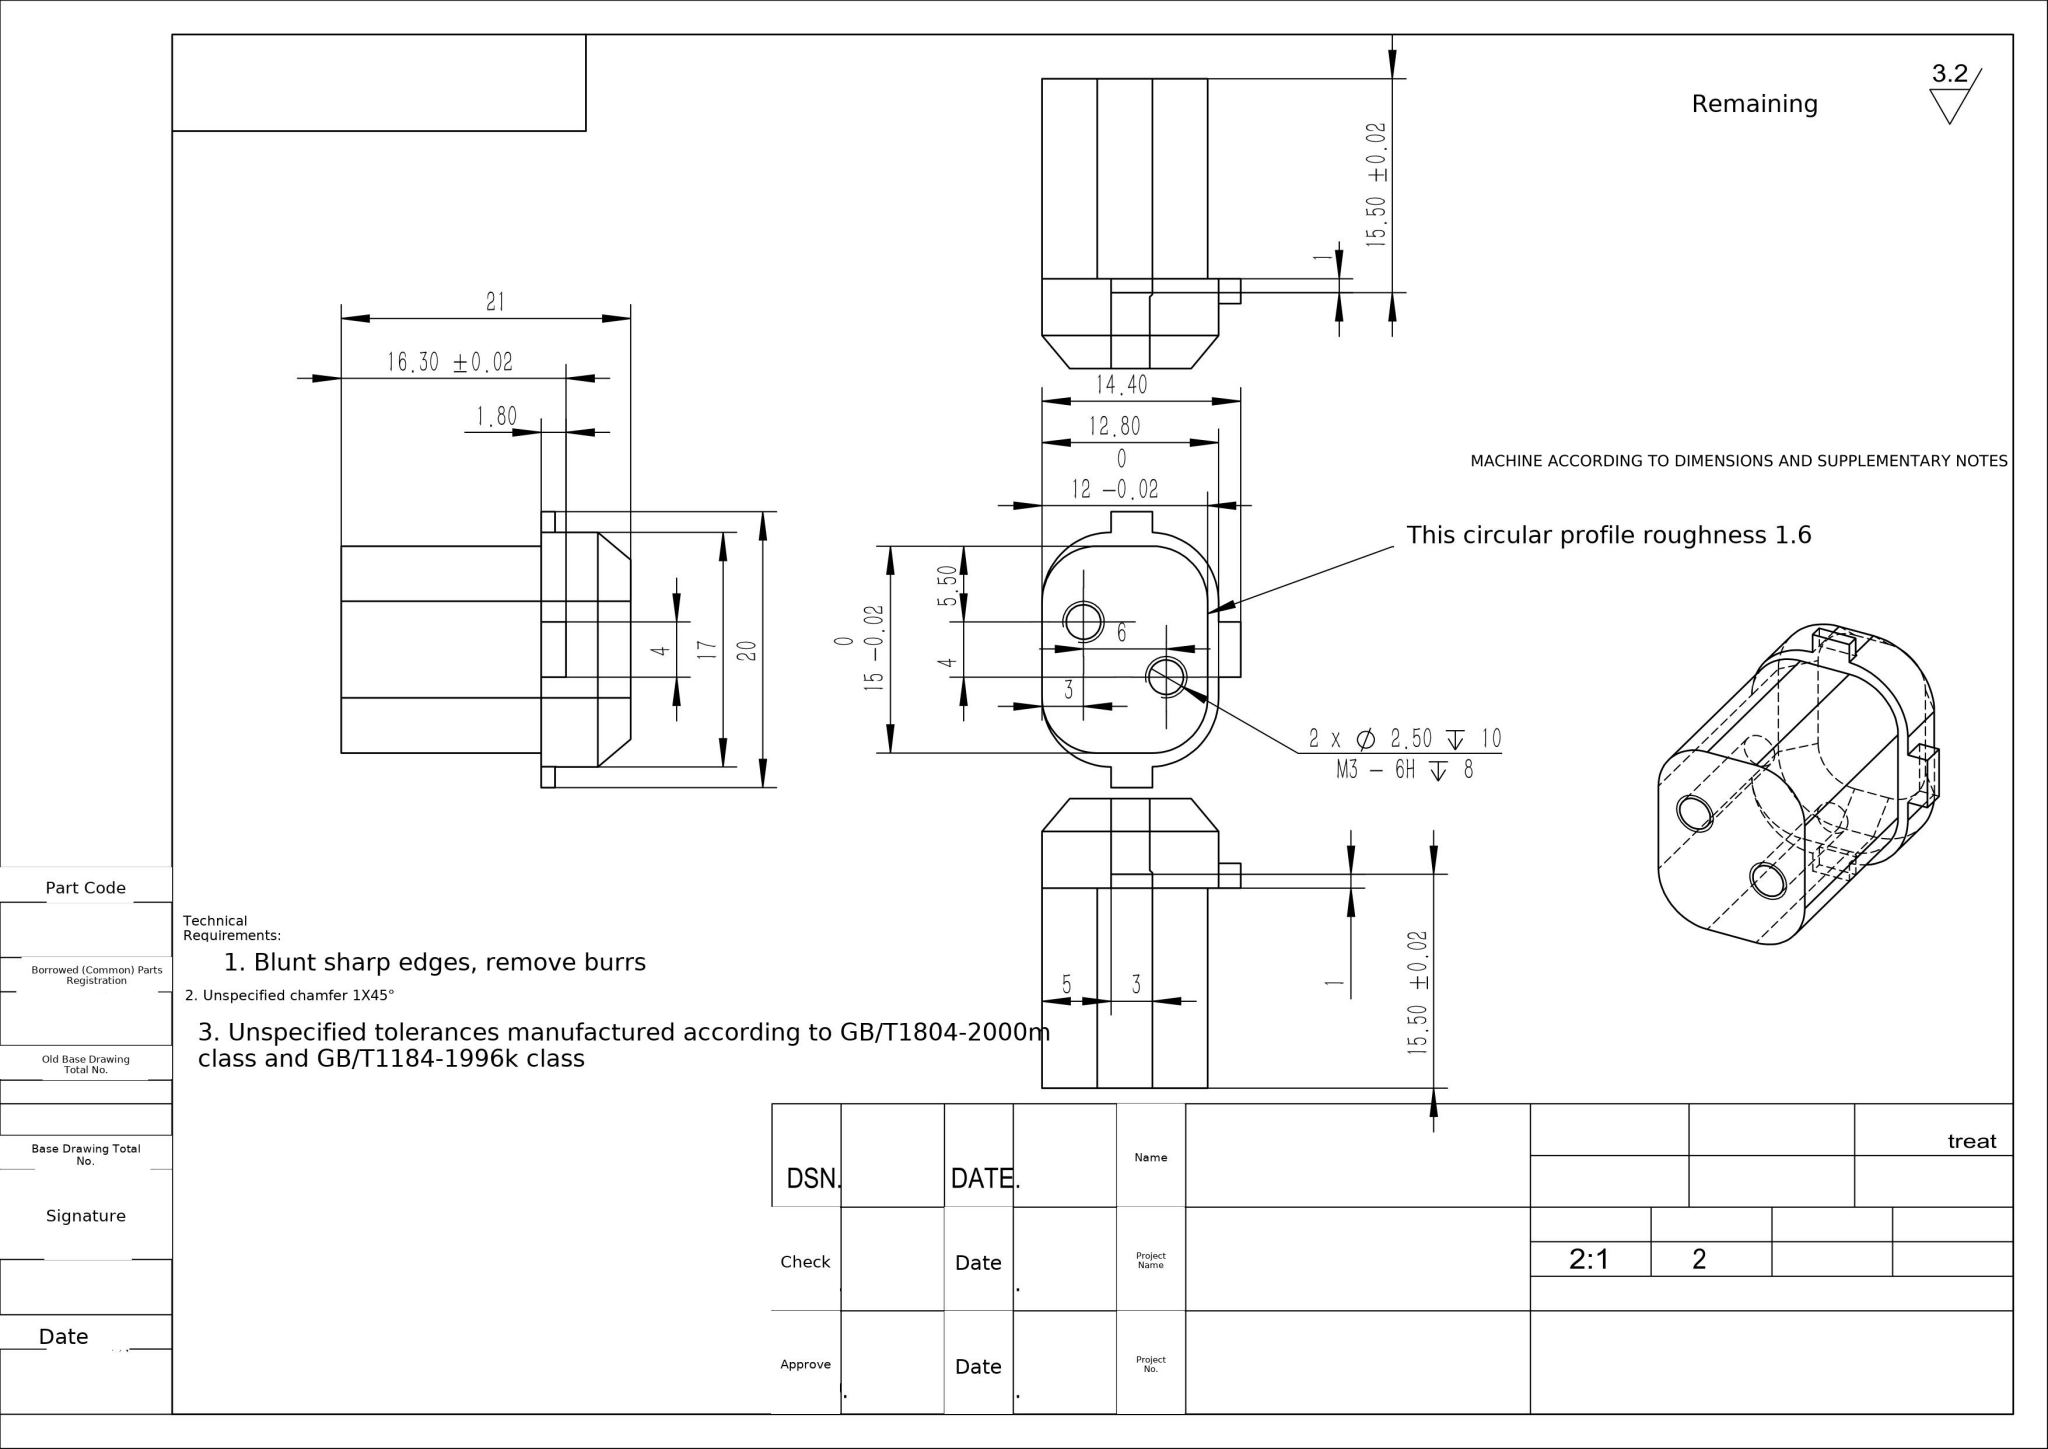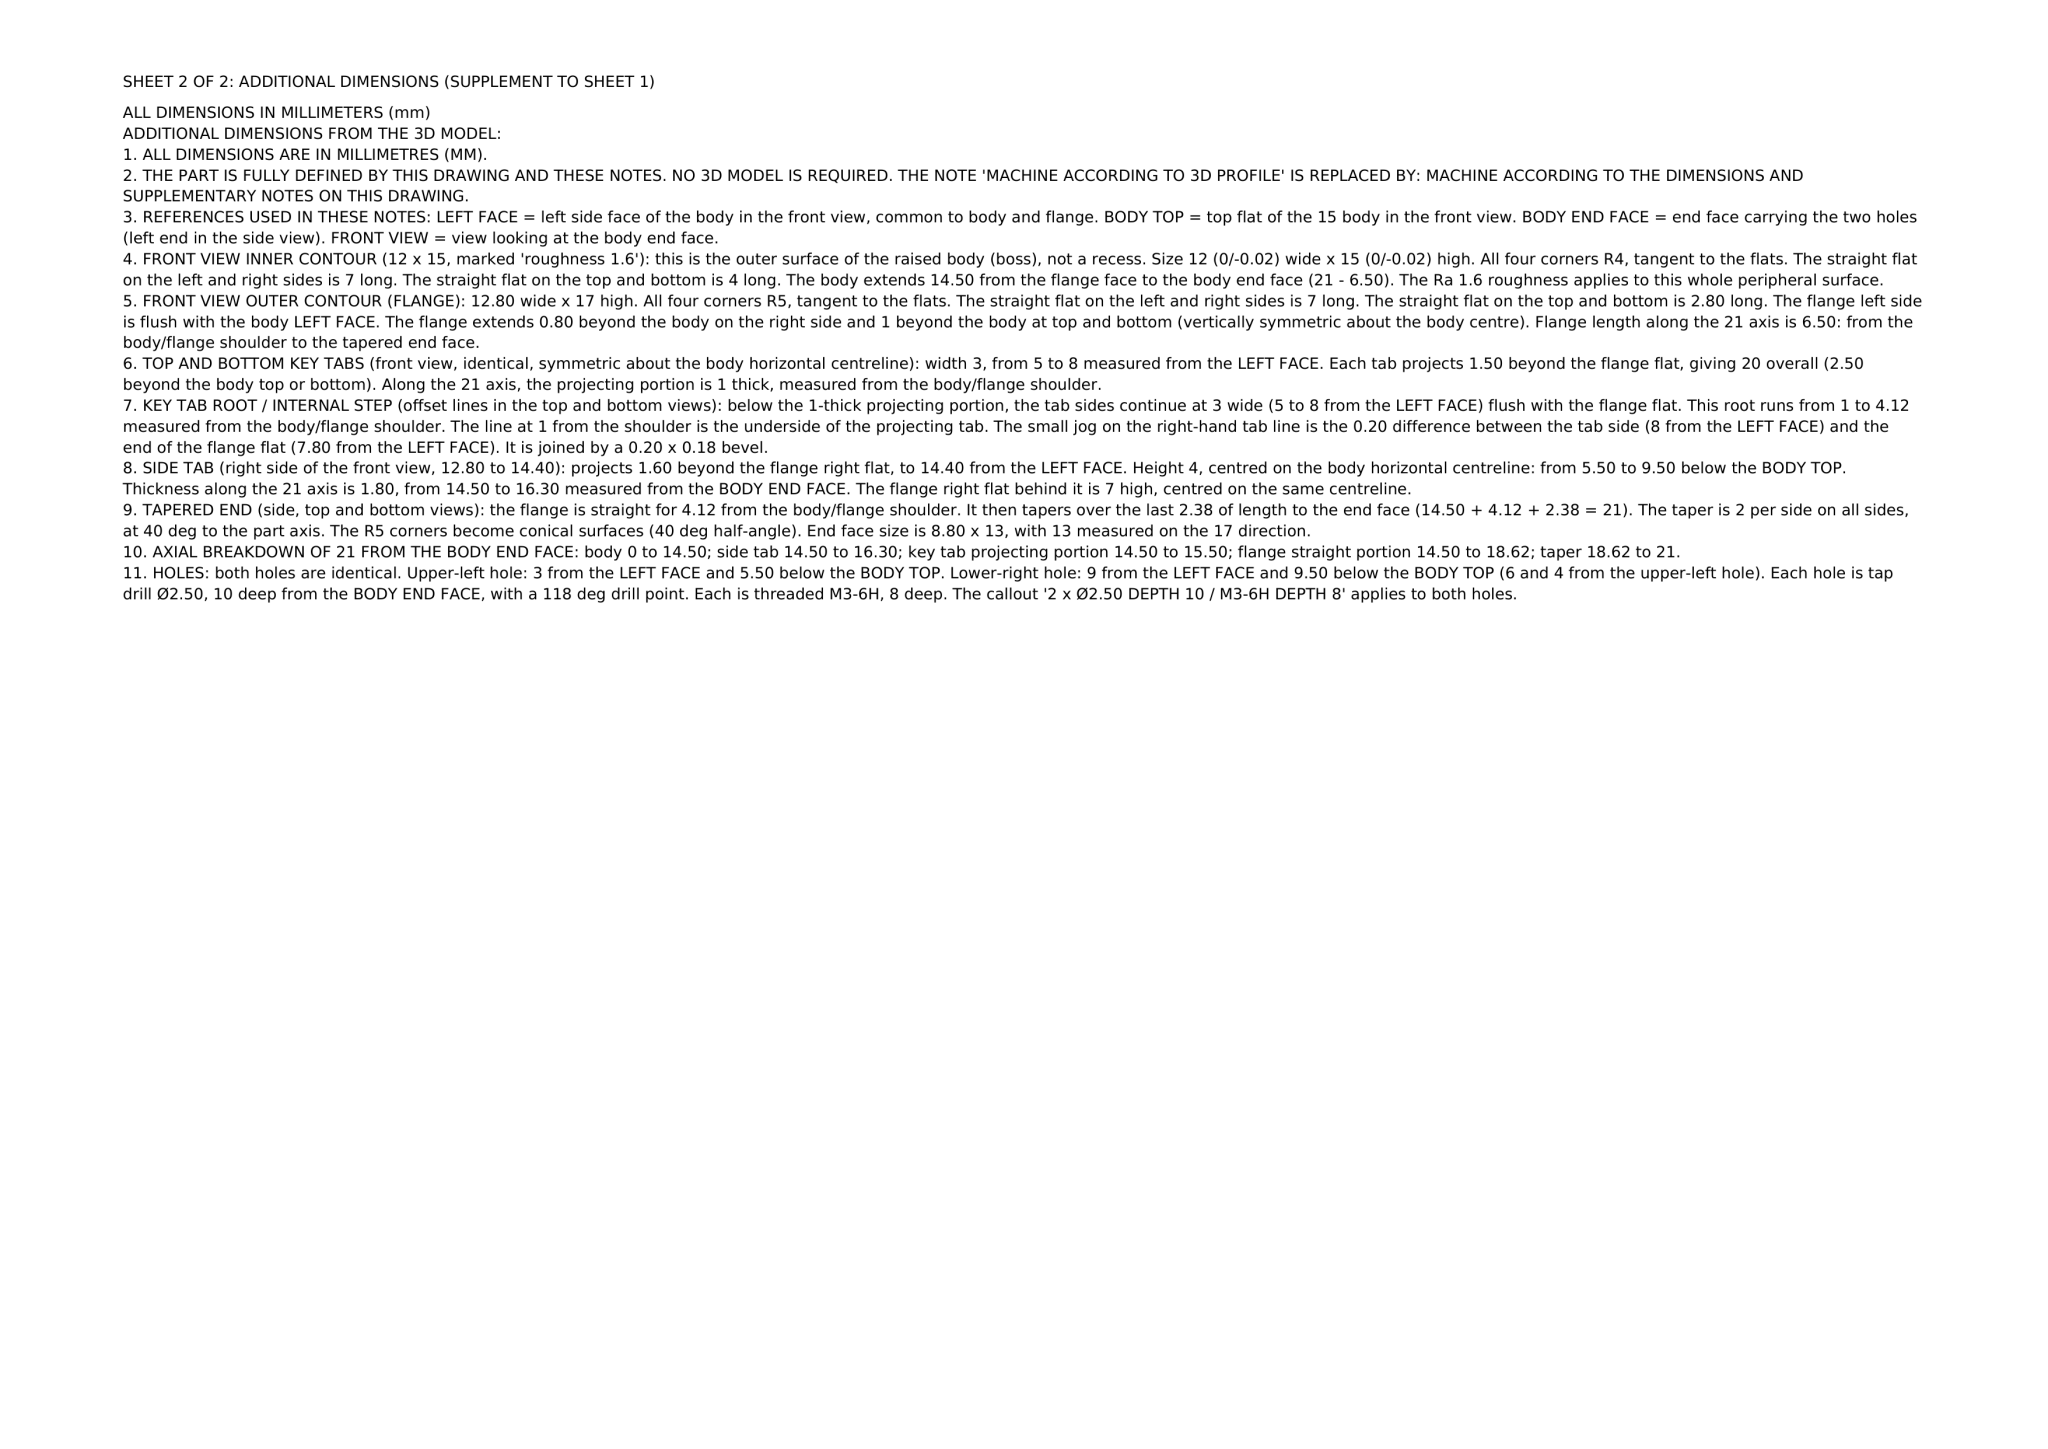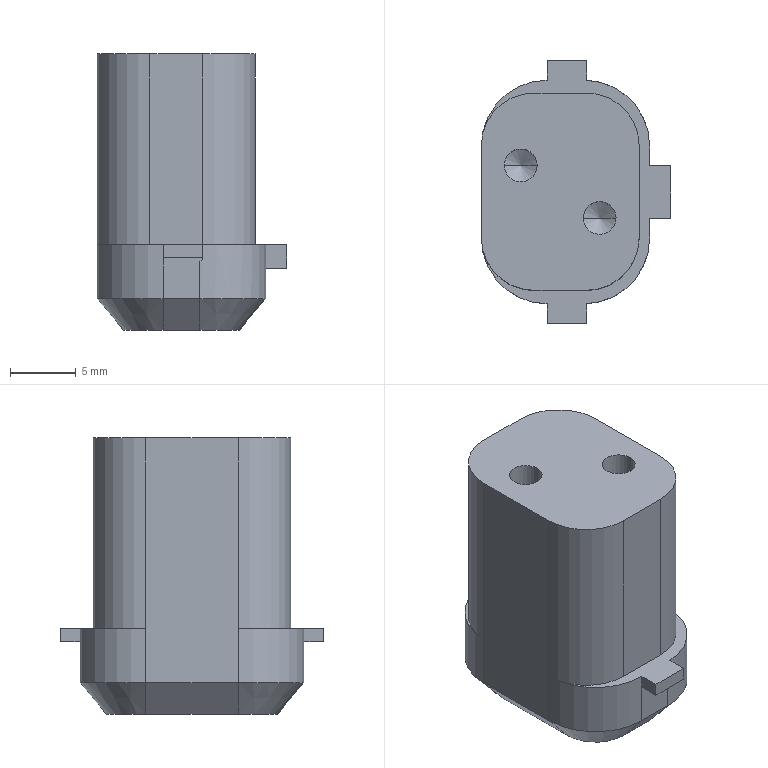Part | NX | mm | Flanged Cylindrical Dual-Bore Mounting Block | 1 solid | 48 faces | box 14.4 x 20 x 21 mm | volume 3494 mm3 | plane 28 | cylinder 12 | cone 8 | commonest cylinder face diameters 2.5 x4 10 x4 8 x4